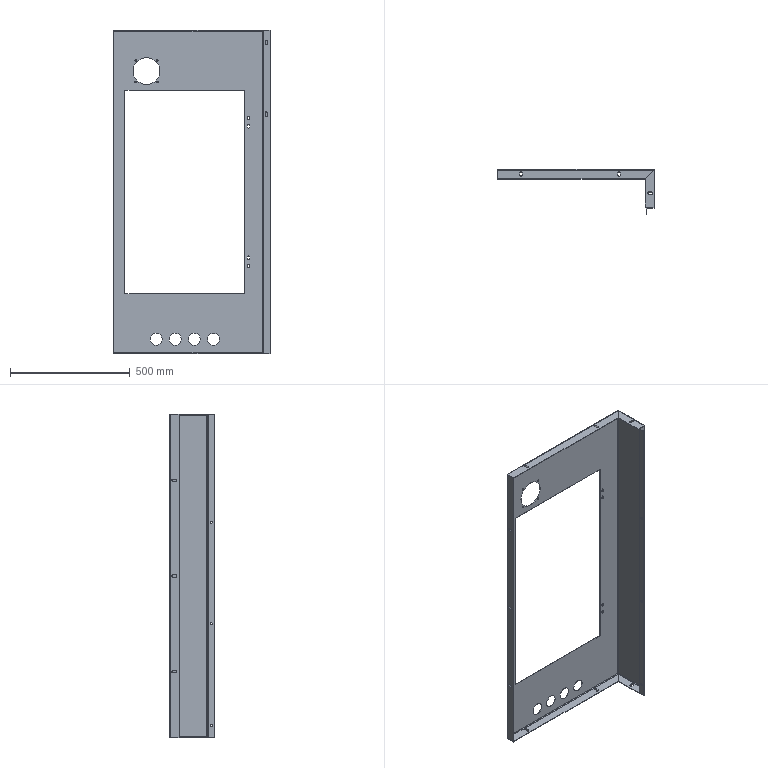Component | SolidWorks | RearRightSidePlateAssembly-1_RearRightSidePlate-1 | 1 solid | 176 faces | volume 1689821 mm3 | plane 88 | cylinder 80 | spline 8 | commonest cylinder face diameters 10 x28 9 x18 50 x8 7 x8 4 x8 8 x8 112 x2 | material Plain Carbon Steel